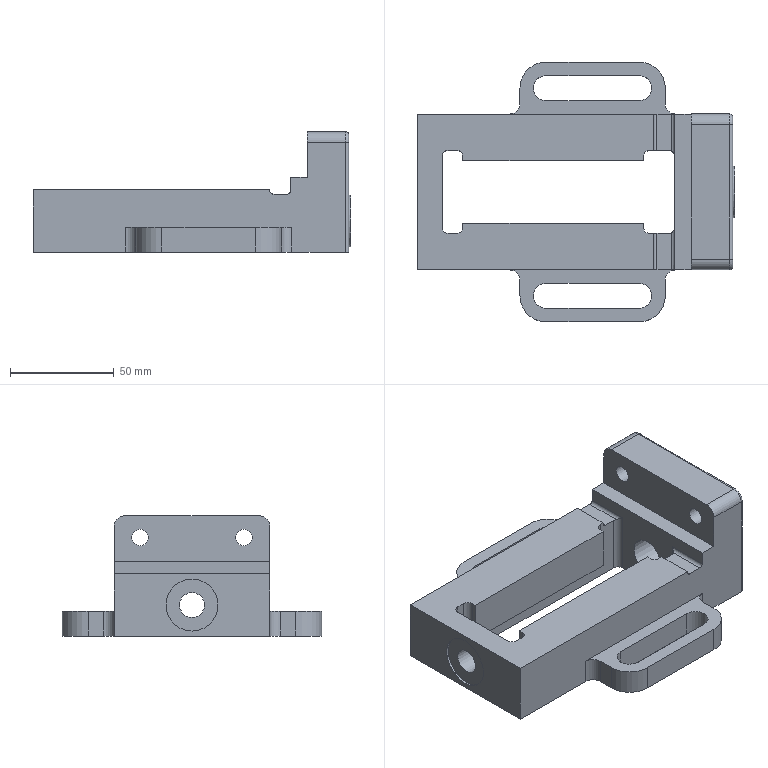Component | NX | 1 | 1 solid | 76 faces | volume 284349 mm3 | plane 39 | cylinder 35 | torus 2 | commonest cylinder face diameters 6 x8 3 x7 25 x6 10 x6 12 x5 8 x2 18 x1